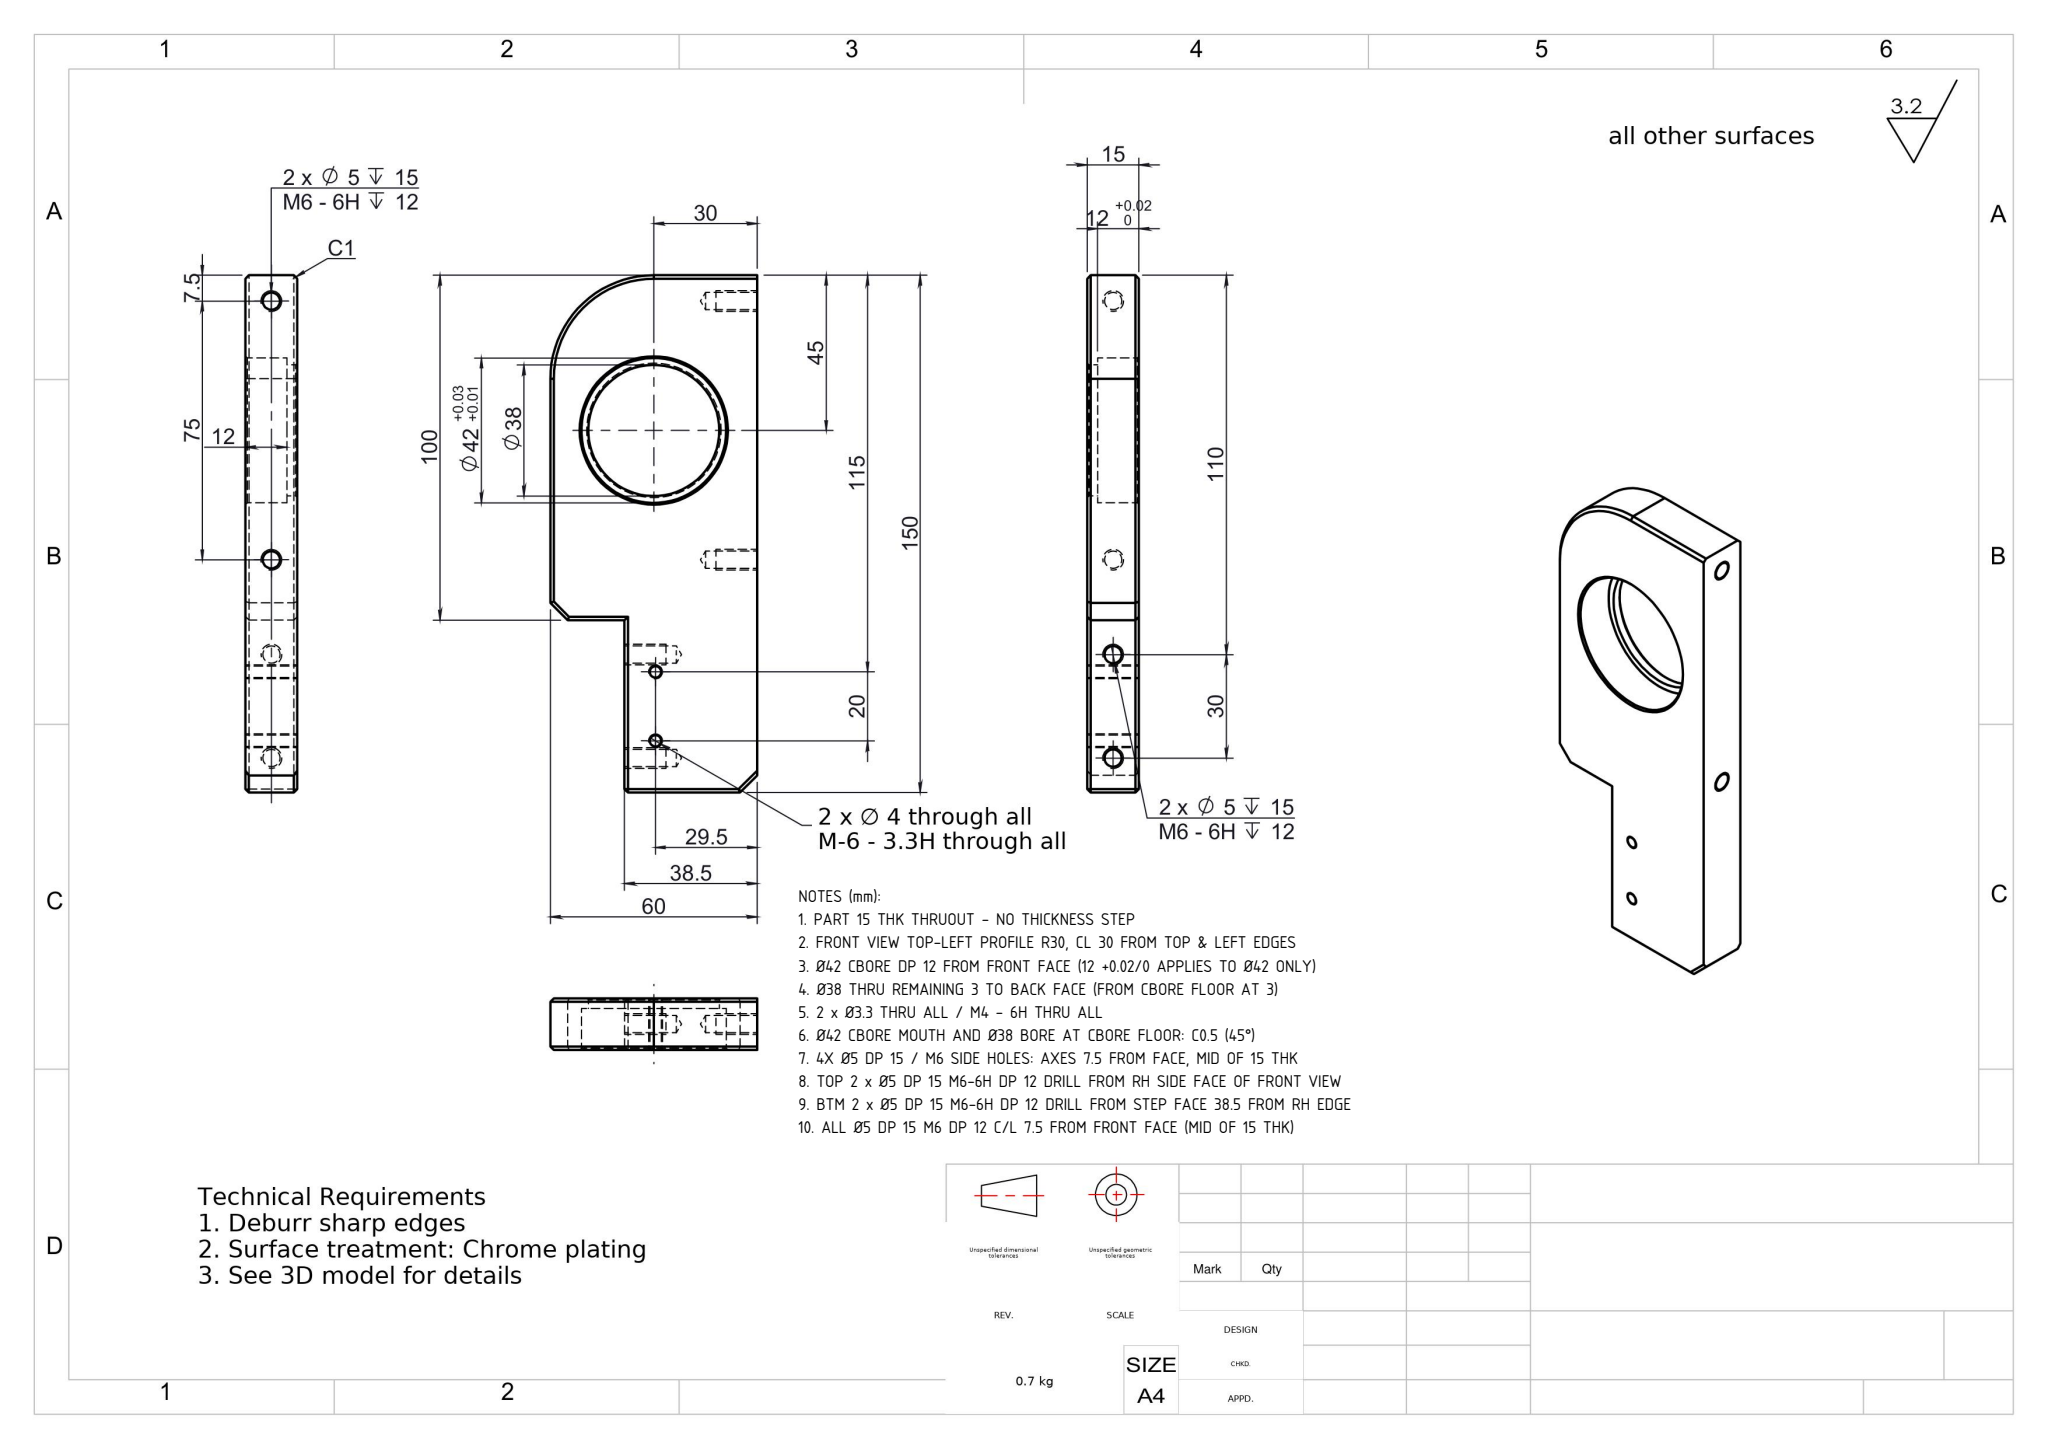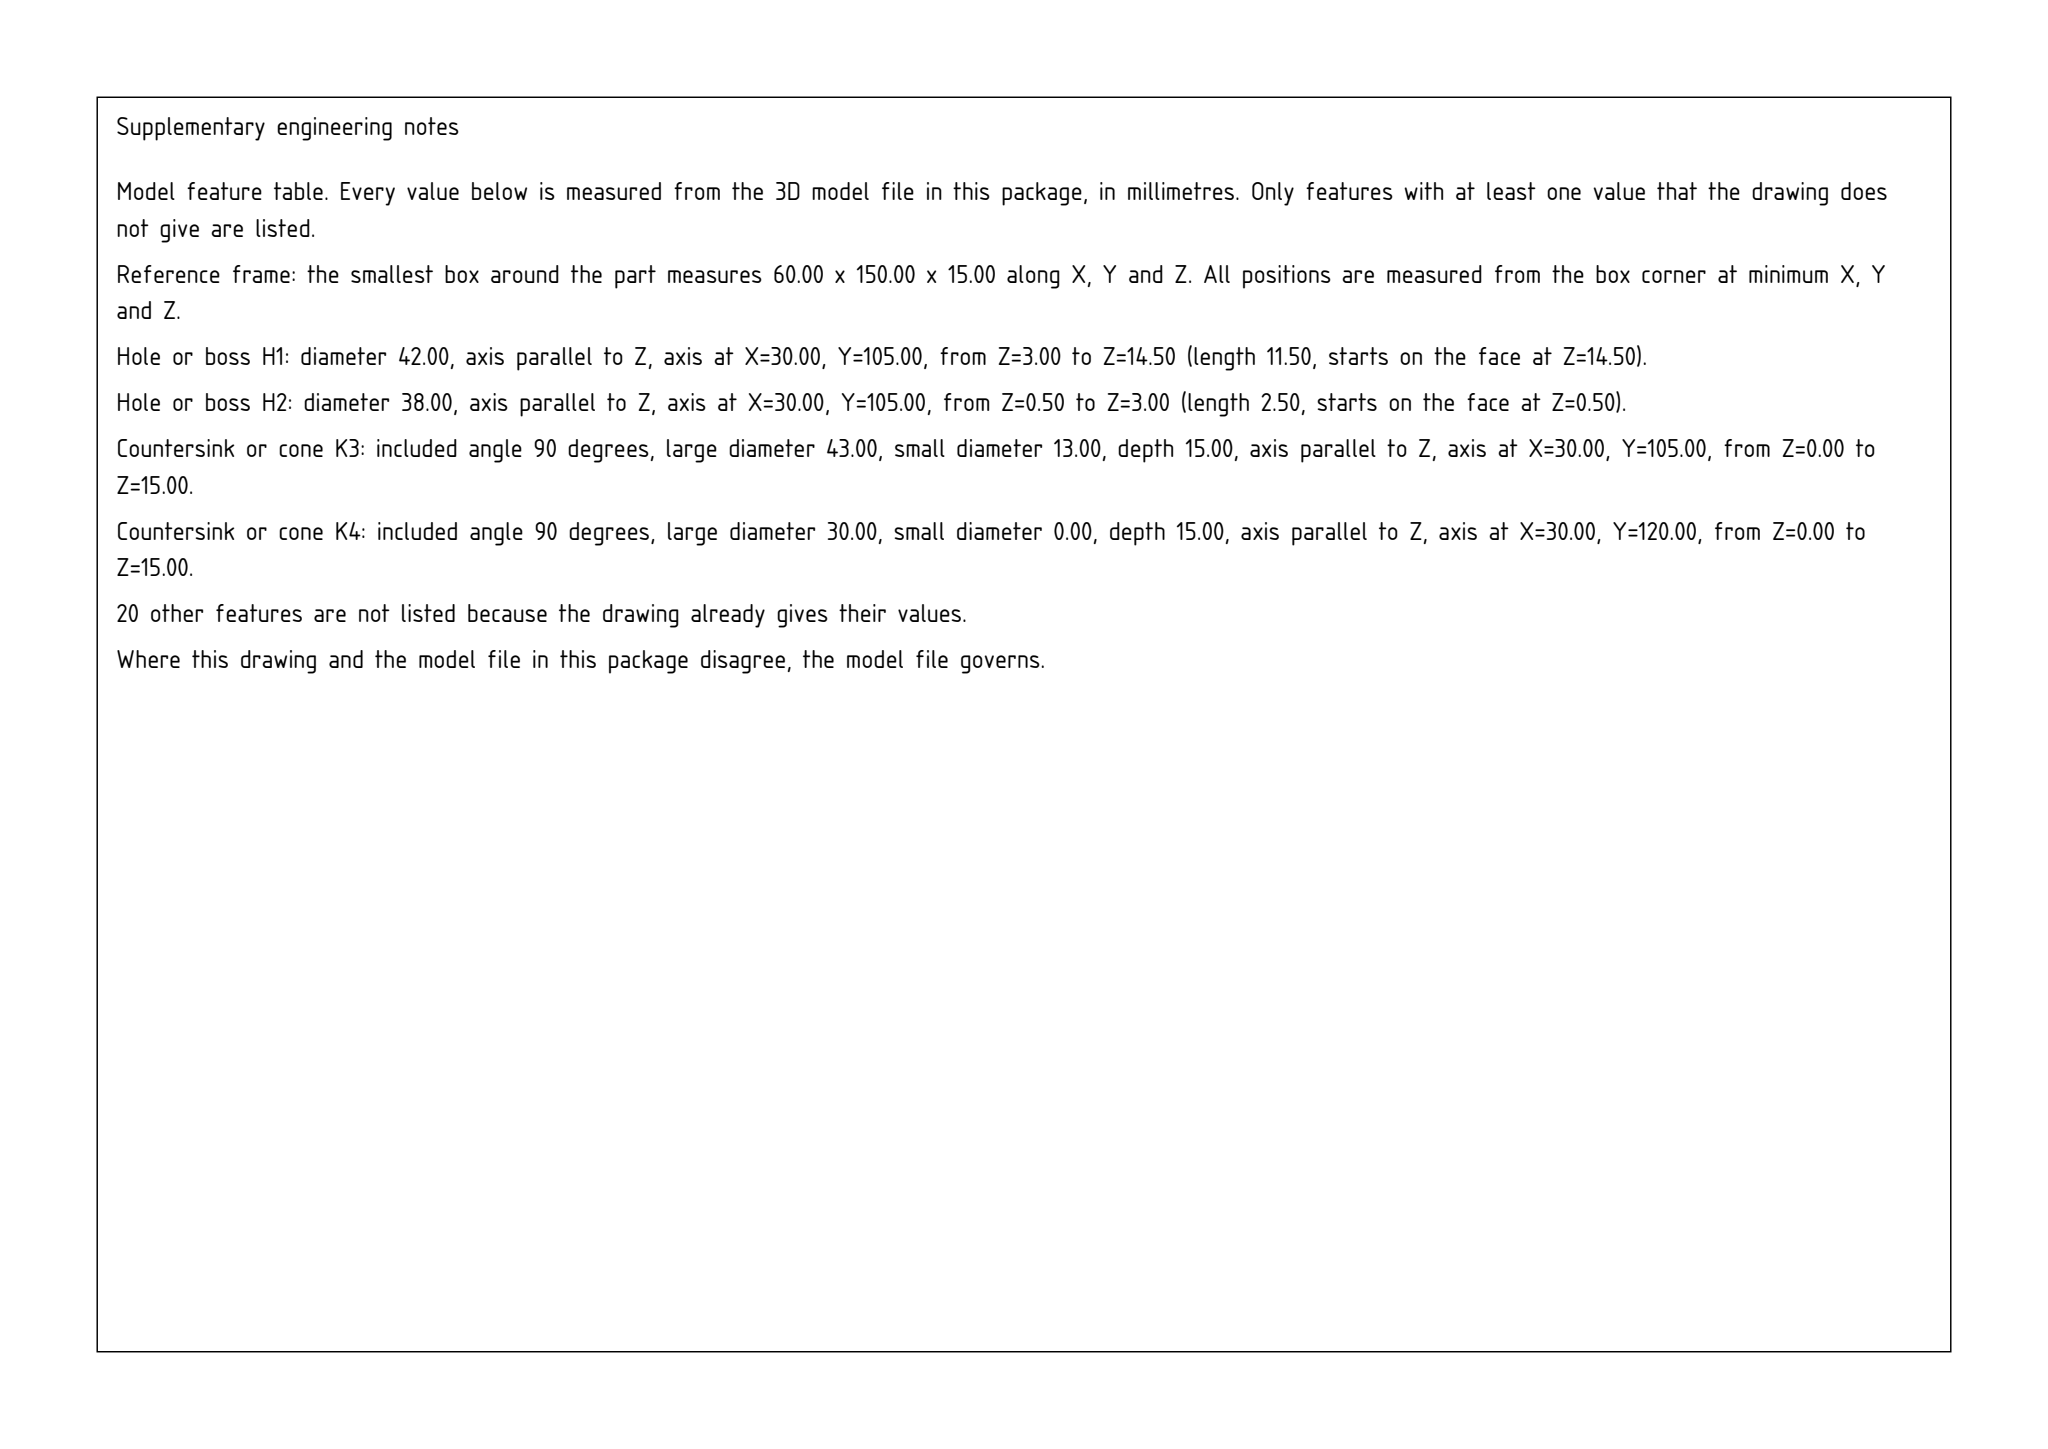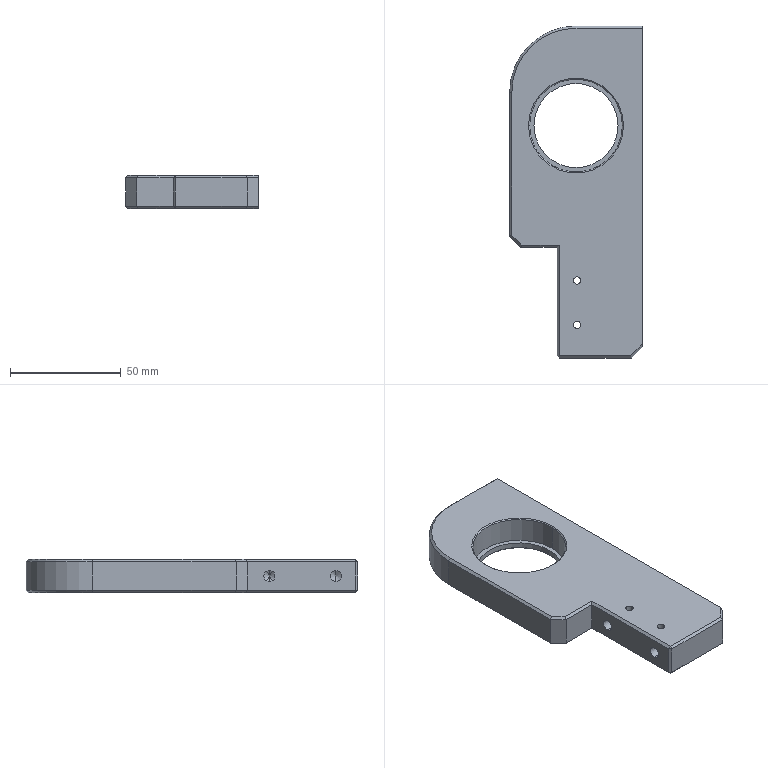Part | SolidWorks | mm | 1 solid | 59 faces | box 60 x 150 x 15 mm | volume 93807 mm3 | plane 28 | cylinder 17 | cone 14 | commonest cylinder face diameters 5 x8 3.3 x4 38 x2 42 x2 60 x1
Drawing notes:
PART 15 THK THRUOUT - NO THICKNESS STEP | from the solid: z planes only 0, 3, 15; Ø3.3 and Ø5 holes full 15 deep -> uniform 15 thk
FRONT VIEW TOP-LEFT PROFILE R30, CL 30 FROM TOP & LEFT EDGES | from the solid: cyl dia 60 about z at (x=30, y=120) -> R30 tangent to top y=150 and left x=0
Ø42 CBORE DP 12 FROM FRONT FACE (12 +0.02/0 APPLIES TO Ø42 ONLY) | from the solid: Ø42 cyl len 11.5 + 90° cone ref Ø42 (1.0) = 12 from z=15 face, floor at z=3
Ø38 THRU REMAINING 3 TO BACK FACE (FROM CBORE FLOOR AT 3) | from the solid: Ø38 cyl len 2.5 + 90° cone ref Ø39 (0.5) = 3 from z=0 face; 12 + 3 = 15
2 x Ø3.3 THRU ALL / M4 - 6H THRU ALL | from the solid: cyls dia 3.3 axis z at (30.5,15) & (30.5,35), len 15 = full thk; 118° drill points
Ø42 CBORE MOUTH AND Ø38 BORE AT CBORE FLOOR: C0.5 (45°) | from the solid: cones 90° incl at ref dia 42 (42->43) and ref dia 39 (38->39) => 0.5 x 45 chamfers on Ø42 cbore mouth and Ø38 bore edge
4X Ø5 DP 15 / M6 SIDE HOLES: AXES 7.5 FROM FACE, MID OF 15 THK | from the solid: cylinders dia 5, axis x, pos z=7.5 (y=10,40,67.5,142.5); bbox z = 15, so axes at mid-thickness
TOP 2 x Ø5 DP 15 M6-6H DP 12 DRILL FROM RH SIDE FACE OF FRONT VIEW | from the solid: Ø5 x-axis holes at Y=67.5 & 142.5, Z=7.5, L=15 entering X=60 face (bbox X=0-60)
BTM 2 x Ø5 DP 15 M6-6H DP 12 DRILL FROM STEP FACE 38.5 FROM RH EDGE | from the solid: Ø5 x-axis holes at Y=10 & 40, Z=7.5, L=15 entering plane x=21.5 (=60-38.5) step face
ALL Ø5 DP 15 M6 DP 12 C/L 7.5 FROM FRONT FACE (MID OF 15 THK) | from the solid: Ø5 cylinders pos z=7.5, part thickness 15 (planes z=0 & z=15)
build123d program:
from build123d import *

# Parameters (mm, degrees)
SKETCH1_W             = 60
SKETCH1_H             = 150
BOSS_EXTRUDE1_DEPTH   = 7.5
SKETCH2_W             = 21.5
SKETCH2_H             = 50
CUT_EXTRUDE1_DEPTH    = 83.158
SKETCH3_R             = 21
CUT_EXTRUDE2_DEPTH    = 12
SKETCH4_R             = 19
CUT_EXTRUDE3_DEPTH    = 82.664
CHAMFER1_SIZE         = 5
M6_TAPPED_HOLE1_D     = 5
M6_TAPPED_HOLE1_DEPTH = 15
M6_TAPPED_HOLE1_TIP   = 1.502
FILLET1_R             = 30
M6_TAPPED_HOLE2_D     = 5
M6_TAPPED_HOLE2_DEPTH = 15
M6_TAPPED_HOLE2_TIP   = 1.502
CHAMFER4_SIZE         = 5
CHAMFER2_SIZE         = 1
CHAMFER3_SIZE         = 0.5
M4_TAPPED_HOLE1_D     = 3.3


with BuildPart() as part:
    # Sketch1 → Boss-Extrude1 (new, symmetric)
    with BuildSketch(Plane.XY):
        Rectangle(SKETCH1_W, SKETCH1_H)
    extrude(amount=BOSS_EXTRUDE1_DEPTH, both=True)

    # Sketch2 → Cut-Extrude1 (cut, through all)
    with BuildSketch(Plane.XY.offset(7.5)):
        with Locations((-19.25, -50)):
            Rectangle(SKETCH2_W, SKETCH2_H)
    extrude(amount=-CUT_EXTRUDE1_DEPTH, mode=Mode.SUBTRACT)

    # Sketch3 → Cut-Extrude2 (cut)
    with BuildSketch(Plane.XY.offset(7.5)):
        with Locations((0, 30)):
            Circle(SKETCH3_R)
    extrude(amount=-CUT_EXTRUDE2_DEPTH, mode=Mode.SUBTRACT)

    # Sketch4 → Cut-Extrude3 (cut, through all)
    with BuildSketch(Plane.XY.offset(-4.5)):
        with Locations((0, 30)):
            Circle(SKETCH4_R)
    extrude(amount=-CUT_EXTRUDE3_DEPTH, mode=Mode.SUBTRACT)

    # Chamfer1
    chamfer1_edges = [part.edges().sort_by_distance(p)[0] for p in [
        (-30, -25, 0),
    ]]
    chamfer(chamfer1_edges, length=CHAMFER1_SIZE)

    # M6 Tapped Hole1
    with Locations(Plane.ZY.offset(8.5)):
        with Locations((0, -35), (0, -65)):
            Hole(M6_TAPPED_HOLE1_D / 2, depth=M6_TAPPED_HOLE1_DEPTH)
            with Locations((0, 0, -(M6_TAPPED_HOLE1_DEPTH + M6_TAPPED_HOLE1_TIP / 2))):  # 118° drill point
                Cone(0, M6_TAPPED_HOLE1_D / 2, M6_TAPPED_HOLE1_TIP, mode=Mode.SUBTRACT)

    # Fillet1
    fillet1_edges = [part.edges().sort_by_distance(p)[0] for p in [
        (-30, 75, 0),
    ]]
    fillet(fillet1_edges, radius=FILLET1_R)

    # M6 Tapped Hole2
    with Locations(Plane(origin=(30, 0, 0), x_dir=(0, 0, -1), z_dir=(1, 0, 0))):
        with Locations((0, -7.5), (0, 67.5)):
            Hole(M6_TAPPED_HOLE2_D / 2, depth=M6_TAPPED_HOLE2_DEPTH)
            with Locations((0, 0, -(M6_TAPPED_HOLE2_DEPTH + M6_TAPPED_HOLE2_TIP / 2))):  # 118° drill point
                Cone(0, M6_TAPPED_HOLE2_D / 2, M6_TAPPED_HOLE2_TIP, mode=Mode.SUBTRACT)

    # Chamfer4
    chamfer4_edges = [part.edges().sort_by_distance(p)[0] for p in [
        (30, -75, 0),
    ]]
    chamfer(chamfer4_edges, length=CHAMFER4_SIZE)

    # Chamfer2
    chamfer2_edges = [part.edges().sort_by_distance(p)[0] for p in [
        (8.25, -75, -7.5),
        (8.25, -75, 7.5),
        (-16.75, -25, -7.5),
        (-8.5, -50, -7.5),
        (-8.5, -75, 0),
        (-8.5, -50, 7.5),
        (-16.75, -25, 7.5),
        (-27.5, -22.5, 7.5),
        (-27.5, -22.5, -7.5),
        (-30, 12.5, -7.5),
        (-30, 12.5, 7.5),
        (-21.213, 66.213, -7.5),
        (15, 75, -7.5),
        (-21.213, 66.213, 7.5),
        (27.5, -72.5, -7.5),
        (27.5, -72.5, 7.5),
        (15, 75, 7.5),
    ]]
    chamfer(chamfer2_edges, length=CHAMFER2_SIZE)

    # Chamfer3
    chamfer3_edges = [part.edges().sort_by_distance(p)[0] for p in [
        (-21, 30, 7.5),
        (-19, 30, -7.5),
    ]]
    chamfer(chamfer3_edges, length=CHAMFER3_SIZE)

    # M4 Tapped Hole1 (through all)
    with Locations(Plane.XY.offset(7.5)):
        with Locations((0.5, -40), (0.5, -60)):
            Hole(M4_TAPPED_HOLE1_D / 2)


solid = part.part